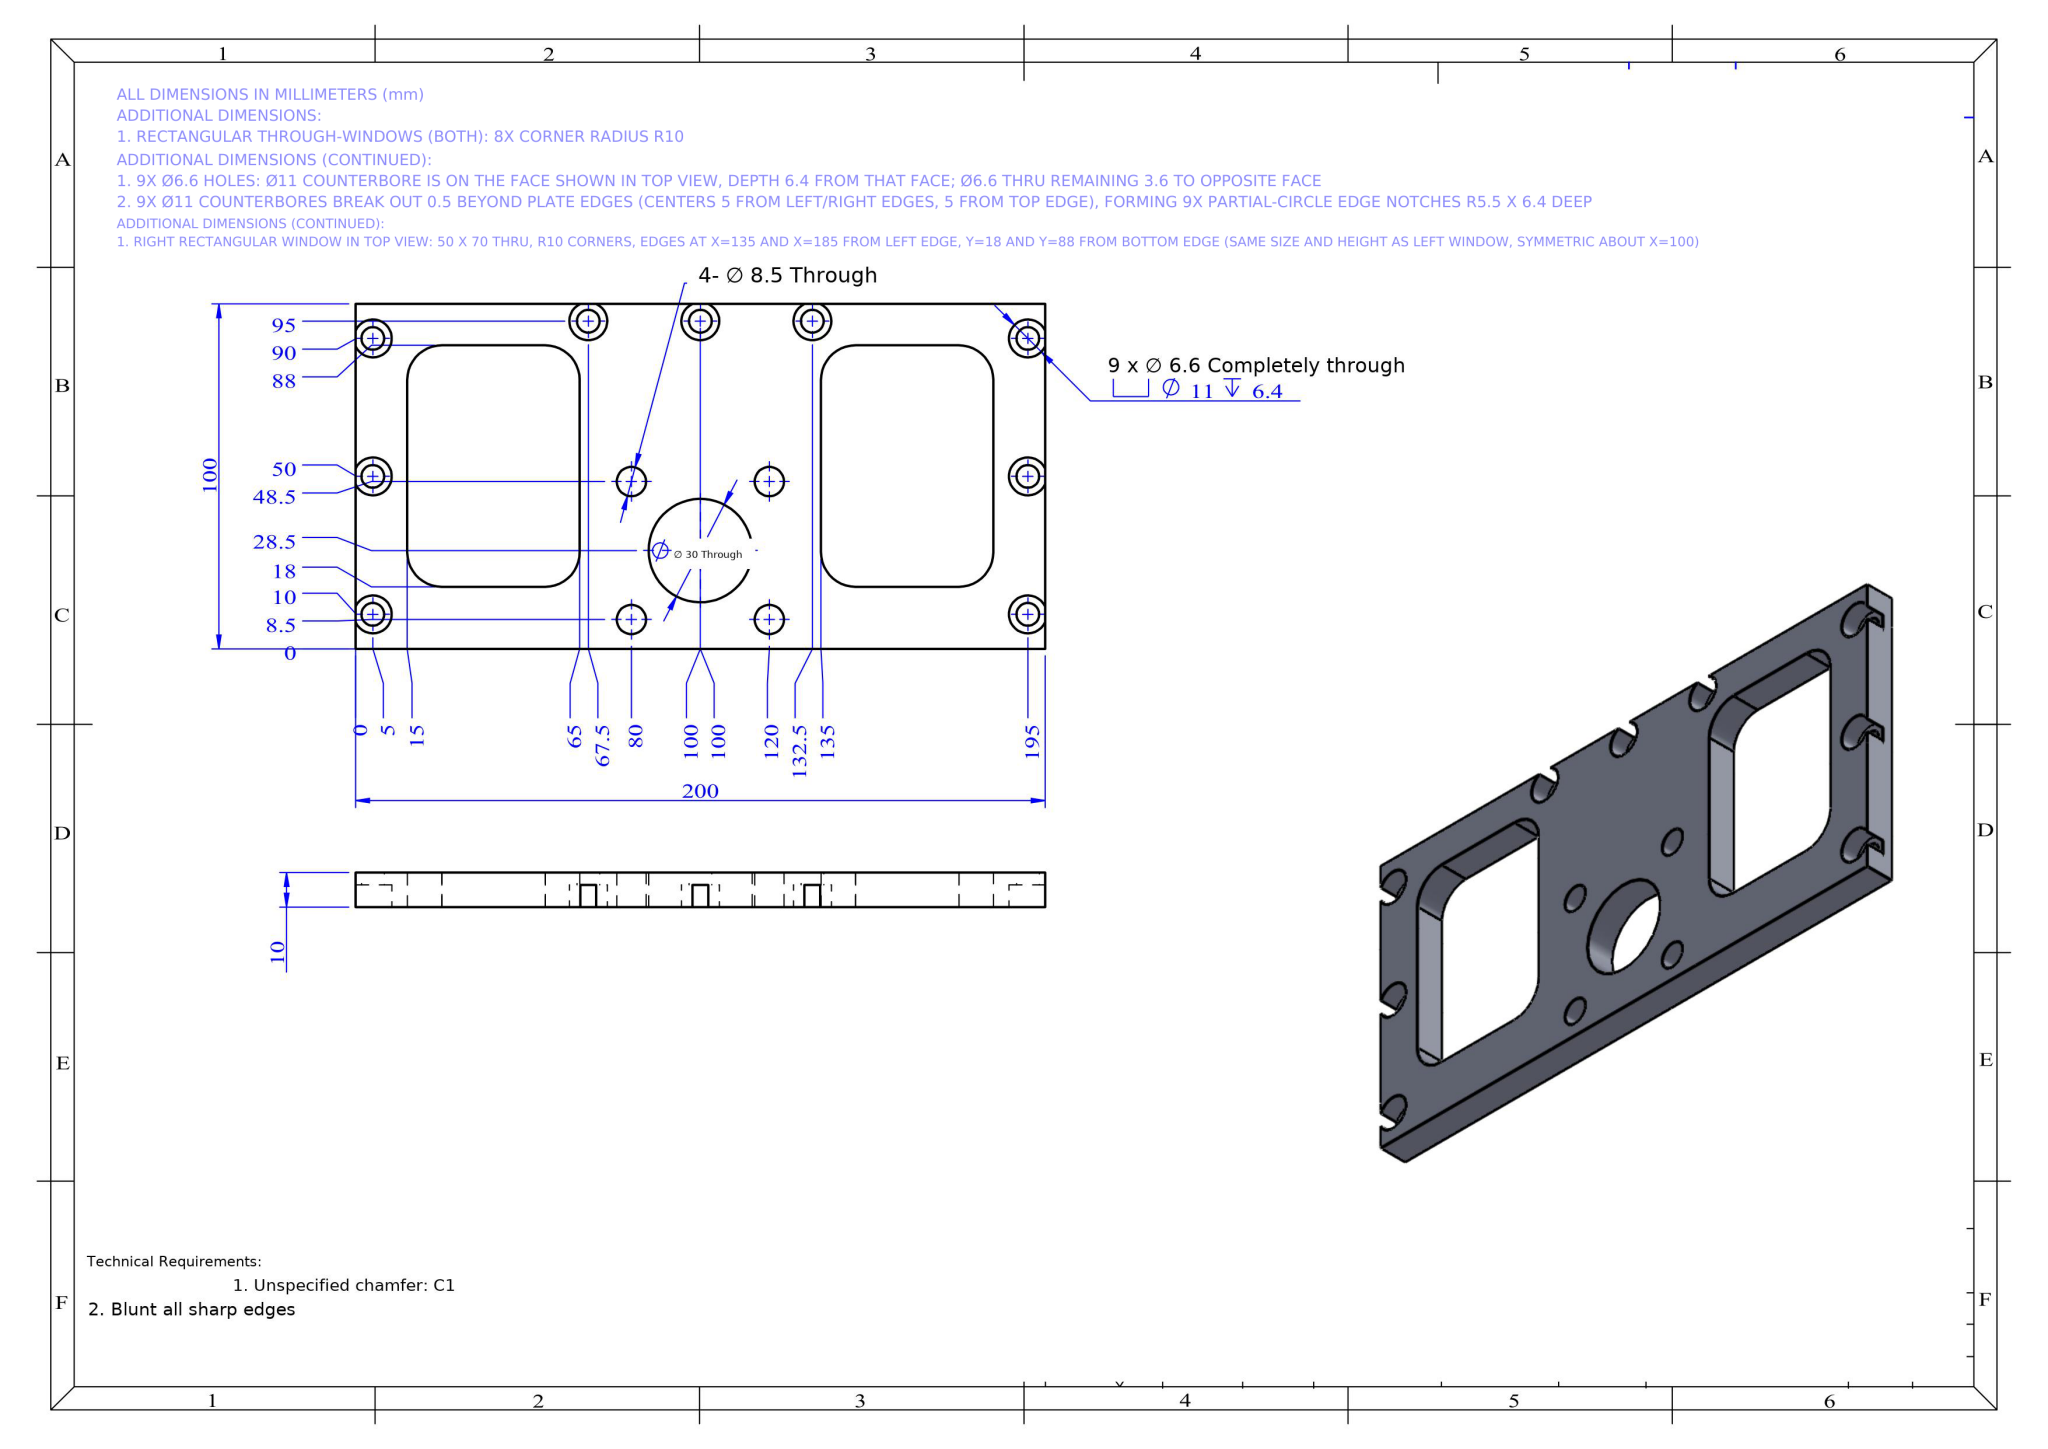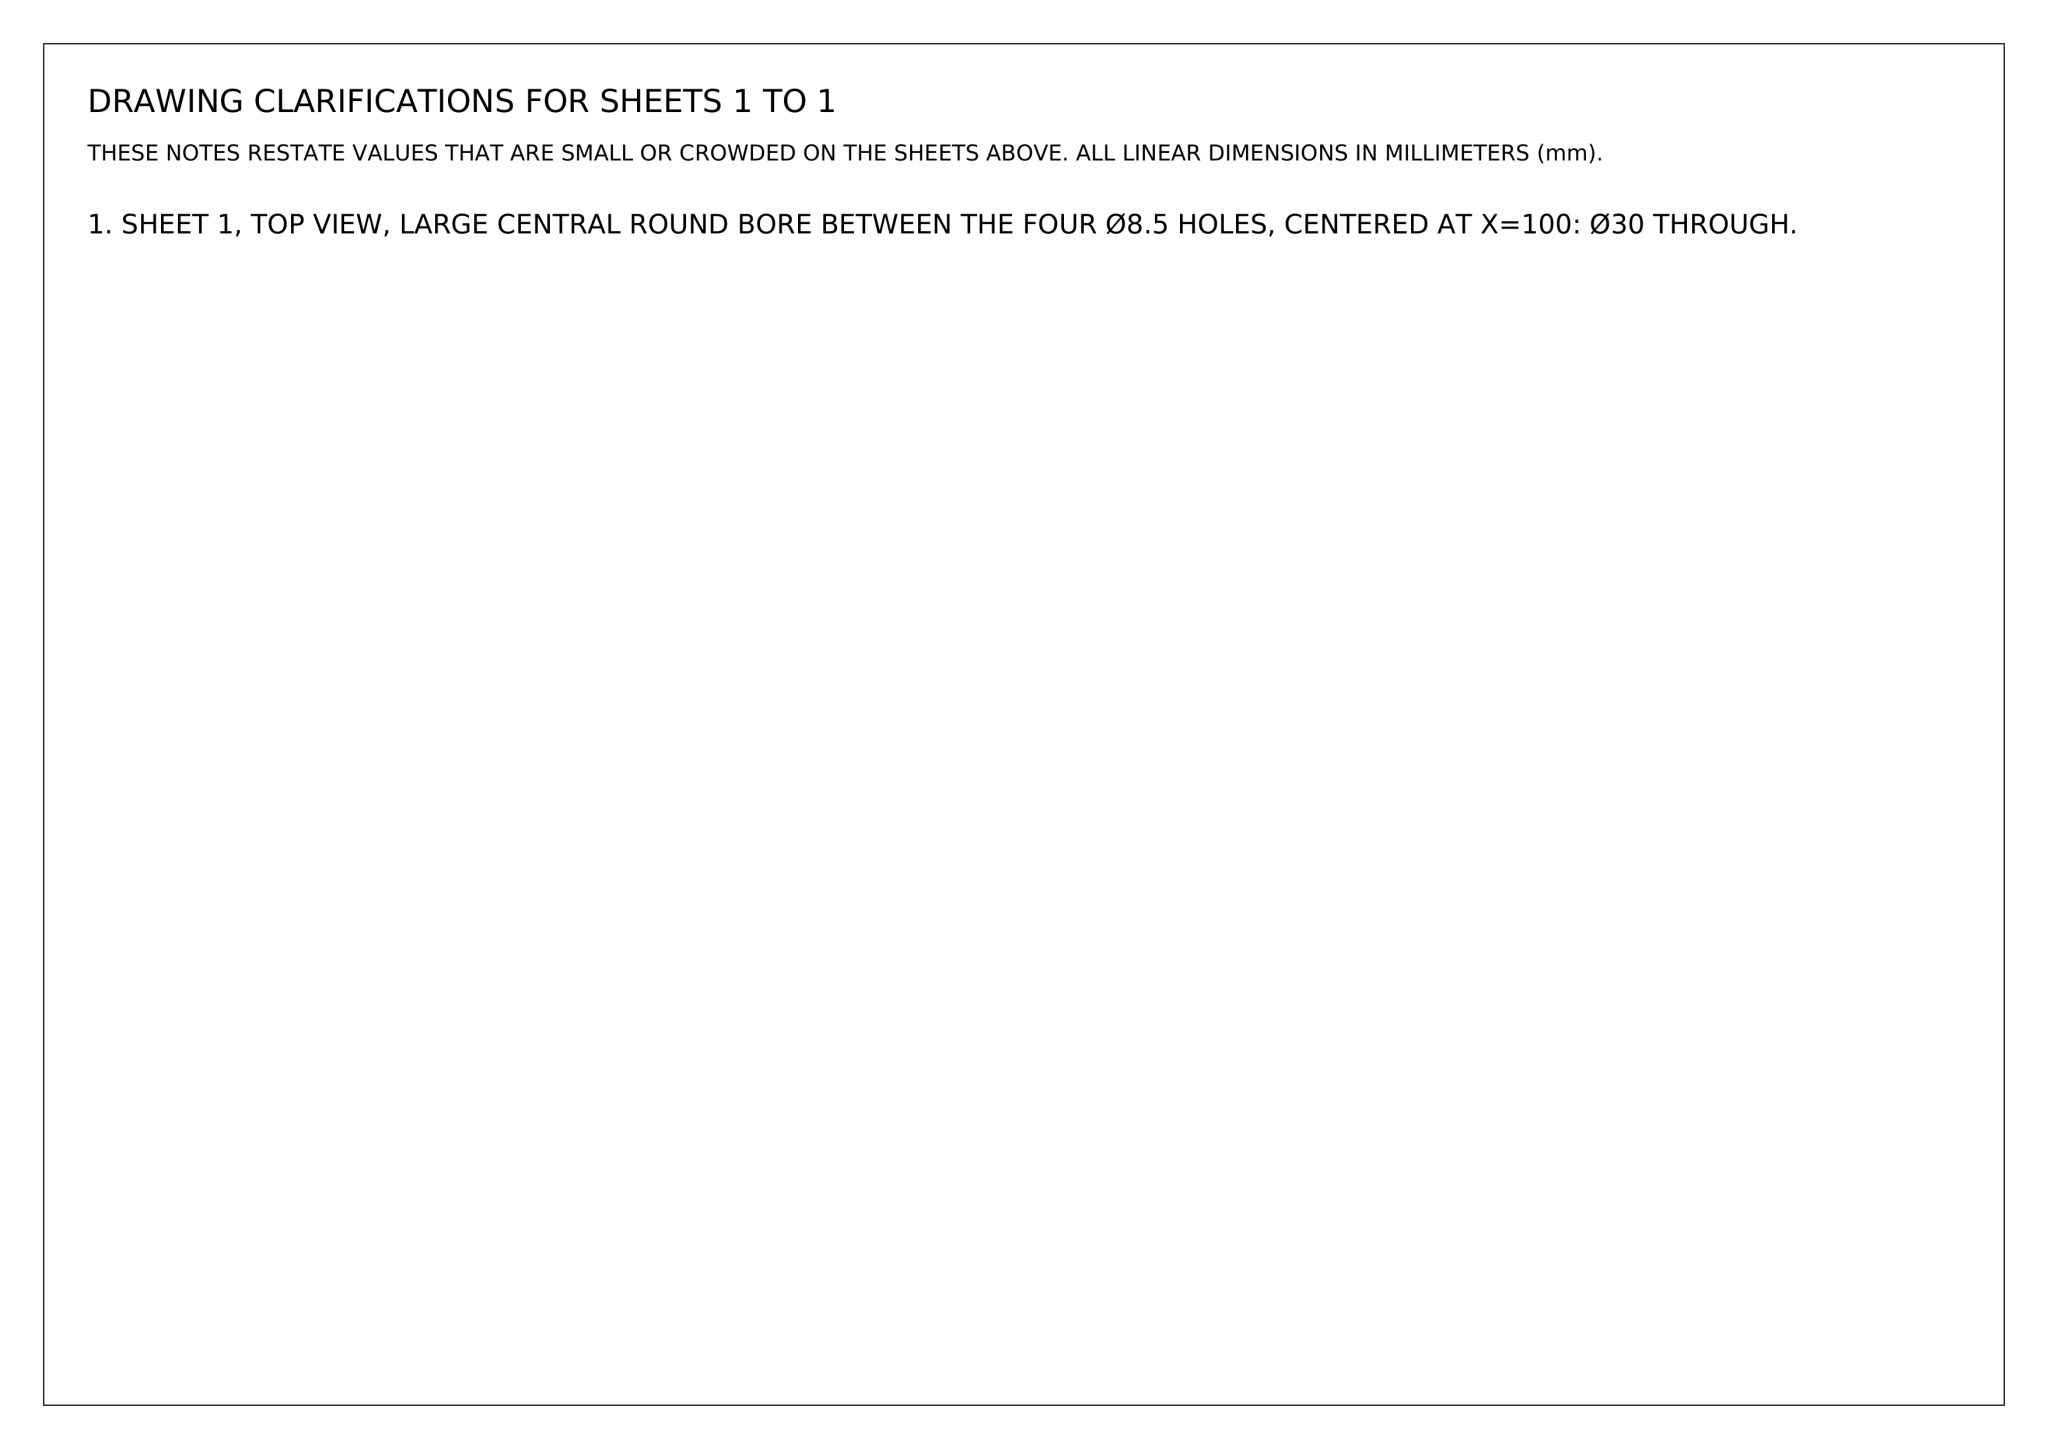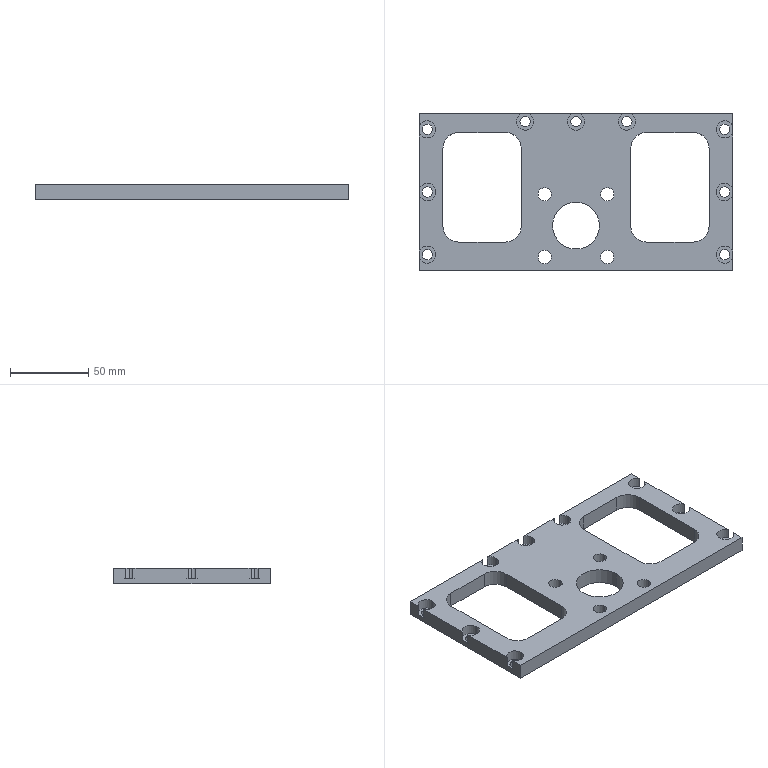Part | NX | mm | 1 solid | 77 faces | box 200 x 100 x 10 mm | volume 115885 mm3 | cylinder 54 | plane 23 | commonest cylinder face diameters 6.6 x18 11 x18 8.5 x8 20 x8 30 x2